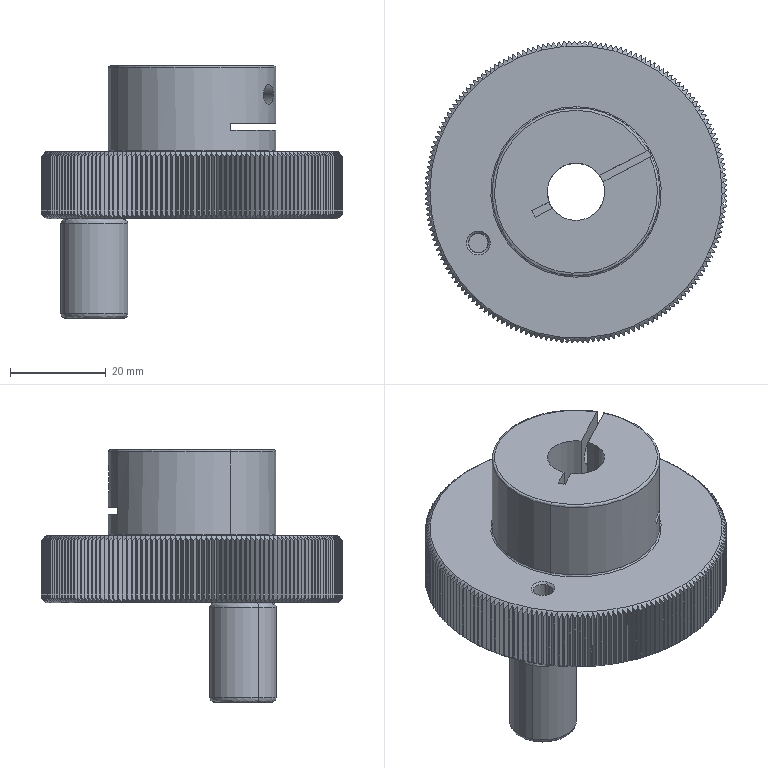Component | SolidWorks | SL010-LeftStreamline-1-1_SL010-2M-0112-000-2-1-1_SL010-HBA41-D63-1-1 | 1 solid | 597 faces | volume 57583 mm3 | plane 383 | cylinder 198 | spline 8 | cone 8 | commonest cylinder face diameters 63 x180 4.134 x4 12 x2 14 x2 35 x2 5.5 x2 10 x2 8.7 x2